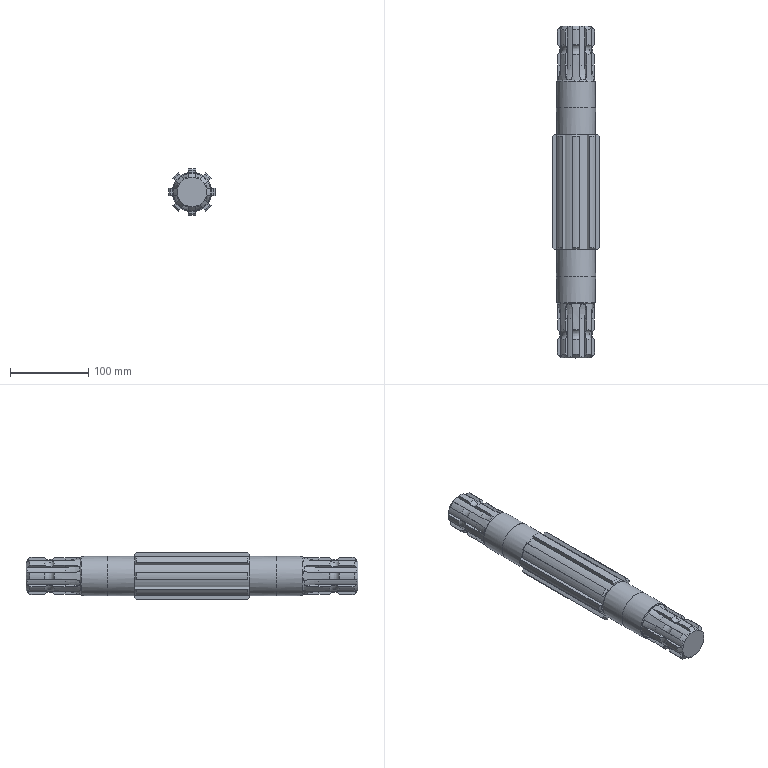Component | NX | SHAFT | 1 solid | 192 faces | volume 834399 mm3 | cylinder 54 | plane 54 | cone 52 | torus 32 | commonest cylinder face diameters 48 x18 40.5 x16 60 x8 50.5 x8 50 x2 49.96 x2